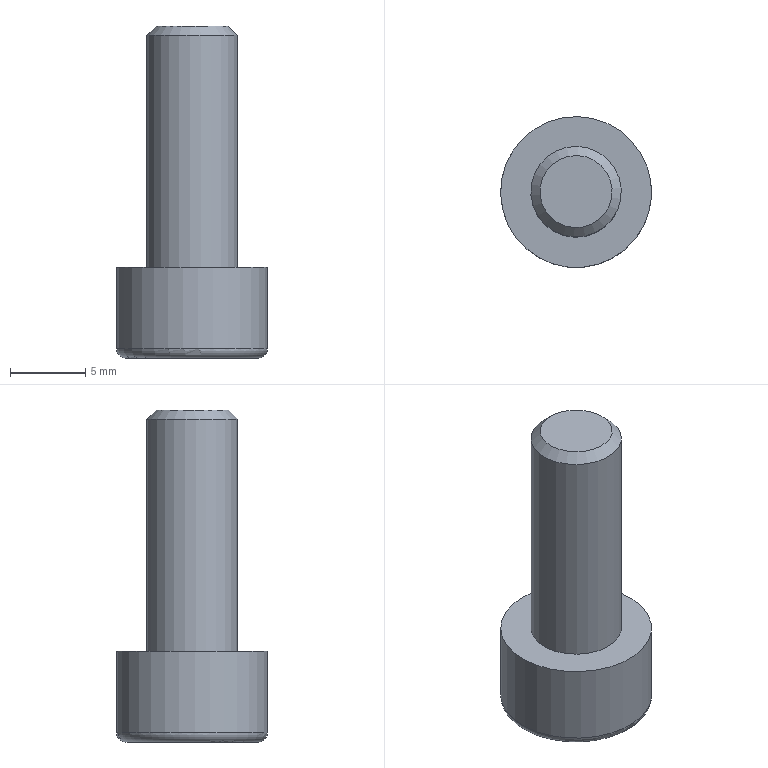Component | NX | SCREW | 1 solid | 14 faces | box 10 x 10 x 22 mm | volume 853 mm3 | plane 10 | cylinder 2 | torus 1 | cone 1 | commonest cylinder face diameters 6 x1 10 x1
STEP:
#1=CARTESIAN_POINT('',(0.,0.,0.));
#2=DIRECTION('',(0.,0.,1.));
#3=DIRECTION('',(1.,0.,0.));
#4=AXIS2_PLACEMENT_3D('',#1,#2,#3);
#5=CARTESIAN_POINT('',(-25.749,-16.598,-131.81));
#6=VERTEX_POINT('',#5);
#7=CARTESIAN_POINT('',(-24.249,-14.,-131.81));
#8=DIRECTION('',(0.,0.,-1.));
#9=DIRECTION('',(-0.5,-0.866,0.));
#10=AXIS2_PLACEMENT_3D('',#7,#8,#9);
#11=CIRCLE('',#10,3.);
#12=CARTESIAN_POINT('',(-24.249,-14.,-147.2));
#13=DIRECTION('',(0.,0.,1.));
#14=DIRECTION('',(0.5,0.866,0.));
#15=AXIS2_PLACEMENT_3D('',#12,#13,#14);
#16=CYLINDRICAL_SURFACE('',#15,3.);
#17=CARTESIAN_POINT('',(9.425,15.39));
#18=DIRECTION('',(-1.,0.));
#19=VECTOR('',#18,1.);
#20=LINE('',#17,#19);
#21=(GEOMETRIC_REPRESENTATION_CONTEXT(2)PARAMETRIC_REPRESENTATION_CONTEXT()REPRESENTATION_CONTEXT('',''));
#22=DEFINITIONAL_REPRESENTATION('',(#20),#21);
#23=PCURVE('',#16,#22);
#24=CARTESIAN_POINT('',(-24.249,-14.,-131.81));
#25=DIRECTION('',(0.,0.,-1.));
#26=DIRECTION('',(-0.5,-0.866,0.));
#27=AXIS2_PLACEMENT_3D('',#24,#25,#26);
#28=CONICAL_SURFACE('',#27,3.,0.7854);
#29=CARTESIAN_POINT('',(0.,0.));
#30=DIRECTION('',(1.,0.));
#31=VECTOR('',#30,1.);
#32=LINE('',#29,#31);
#33=(GEOMETRIC_REPRESENTATION_CONTEXT(2)PARAMETRIC_REPRESENTATION_CONTEXT()REPRESENTATION_CONTEXT('',''));
#34=DEFINITIONAL_REPRESENTATION('',(#32),#33);
#35=PCURVE('',#28,#34);
#36=SURFACE_CURVE('',#11,(#23,#35),.PCURVE_S1.);
#37=EDGE_CURVE('',#6,#6,#36,.T.);
#38=ORIENTED_EDGE('',*,*,#37,.T.);
#39=CARTESIAN_POINT('',(-25.749,-16.598,-147.2));
#40=VERTEX_POINT('',#39);
#41=CARTESIAN_POINT('',(-25.749,-16.598,-147.2));
#42=CARTESIAN_POINT('',(-25.749,-16.598,-131.81));
#43=B_SPLINE_CURVE_WITH_KNOTS('',1,(#41,#42),.UNSPECIFIED.,.F.,.F.,(2,2),(0.,15.39),.PIECEWISE_BEZIER_KNOTS.);
#44=CARTESIAN_POINT('',(3.142,0.));
#45=DIRECTION('',(0.,1.));
#46=VECTOR('',#45,1.);
#47=LINE('',#44,#46);
#48=(GEOMETRIC_REPRESENTATION_CONTEXT(2)PARAMETRIC_REPRESENTATION_CONTEXT()REPRESENTATION_CONTEXT('',''));
#49=DEFINITIONAL_REPRESENTATION('',(#47),#48);
#50=PCURVE('',#16,#49);
#51=CARTESIAN_POINT('',(9.425,0.));
#52=DIRECTION('',(0.,1.));
#53=VECTOR('',#52,1.);
#54=LINE('',#51,#53);
#55=(GEOMETRIC_REPRESENTATION_CONTEXT(2)PARAMETRIC_REPRESENTATION_CONTEXT()REPRESENTATION_CONTEXT('',''));
#56=DEFINITIONAL_REPRESENTATION('',(#54),#55);
#57=PCURVE('',#16,#56);
#58=SEAM_CURVE('',#43,(#50,#57),.PCURVE_S1.);
#59=EDGE_CURVE('',#40,#6,#58,.T.);
#60=ORIENTED_EDGE('',*,*,#59,.F.);
#61=CARTESIAN_POINT('',(-24.249,-14.,-147.2));
#62=DIRECTION('',(0.,0.,-1.));
#63=DIRECTION('',(-0.5,-0.866,0.));
#64=AXIS2_PLACEMENT_3D('',#61,#62,#63);
#65=CIRCLE('',#64,3.);
#66=CARTESIAN_POINT('',(9.425,0.));
#67=DIRECTION('',(-1.,0.));
#68=VECTOR('',#67,1.);
#69=LINE('',#66,#68);
#70=(GEOMETRIC_REPRESENTATION_CONTEXT(2)PARAMETRIC_REPRESENTATION_CONTEXT()REPRESENTATION_CONTEXT('',''));
#71=DEFINITIONAL_REPRESENTATION('',(#69),#70);
#72=PCURVE('',#16,#71);
#73=CARTESIAN_POINT('',(-24.249,-14.,-147.2));
#74=DIRECTION('',(0.,0.,-1.));
#75=DIRECTION('',(-0.5,-0.866,0.));
#76=AXIS2_PLACEMENT_3D('',#73,#74,#75);
#77=PLANE('',#76);
#78=CARTESIAN_POINT('',(0.,0.));
#79=DIRECTION('',(1.,0.));
#80=AXIS2_PLACEMENT_2D('',#78,#79);
#81=CIRCLE('',#80,3.);
#82=(GEOMETRIC_REPRESENTATION_CONTEXT(2)PARAMETRIC_REPRESENTATION_CONTEXT()REPRESENTATION_CONTEXT('',''));
#83=DEFINITIONAL_REPRESENTATION('',(#81),#82);
#84=PCURVE('',#77,#83);
#85=SURFACE_CURVE('',#65,(#72,#84),.PCURVE_S1.);
#86=EDGE_CURVE('',#40,#40,#85,.T.);
#87=ORIENTED_EDGE('',*,*,#86,.F.);
#88=ORIENTED_EDGE('',*,*,#59,.T.);
#89=EDGE_LOOP('',(#38,#60,#87,#88));
#90=FACE_BOUND('',#89,.T.);
#91=ADVANCED_FACE('',(#90),#16,.T.);
#92=CARTESIAN_POINT('',(-25.444,-16.07,-131.2));
#93=VERTEX_POINT('',#92);
#94=CARTESIAN_POINT('',(-24.249,-14.,-131.2));
#95=DIRECTION('',(0.,0.,1.));
#96=DIRECTION('',(-0.5,-0.866,0.));
#97=AXIS2_PLACEMENT_3D('',#94,#95,#96);
#98=CIRCLE('',#97,2.39);
#99=CARTESIAN_POINT('',(-24.249,-14.,-131.2));
#100=DIRECTION('',(0.,0.,-1.));
#101=DIRECTION('',(-0.5,-0.866,0.));
#102=AXIS2_PLACEMENT_3D('',#99,#100,#101);
#103=PLANE('',#102);
#104=CARTESIAN_POINT('',(2.39,0.));
#105=CARTESIAN_POINT('',(2.39,-4.14));
#106=CARTESIAN_POINT('',(-1.195,-2.07));
#107=CARTESIAN_POINT('',(-4.78,-0.));
#108=CARTESIAN_POINT('',(-1.195,2.07));
#109=CARTESIAN_POINT('',(2.39,4.14));
#110=CARTESIAN_POINT('',(2.39,0.));
#111=(BOUNDED_CURVE()B_SPLINE_CURVE(2,(#104,#105,#106,#107,#108,#109,#110),.UNSPECIFIED.,.T.,.F.)B_SPLINE_CURVE_WITH_KNOTS((1,2,2,2,2,1),(-2.094,0.,2.094,4.189,6.283,8.378),.UNSPECIFIED.)CURVE()GEOMETRIC_REPRESENTATION_ITEM()RATIONAL_B_SPLINE_CURVE((1.,0.5,1.,0.5,1.,0.5,1.))REPRESENTATION_ITEM(''));
#112=(GEOMETRIC_REPRESENTATION_CONTEXT(2)PARAMETRIC_REPRESENTATION_CONTEXT()REPRESENTATION_CONTEXT('',''));
#113=DEFINITIONAL_REPRESENTATION('',(#111),#112);
#114=PCURVE('',#103,#113);
#115=CARTESIAN_POINT('',(6.283,-0.61));
#116=DIRECTION('',(-1.,0.));
#117=VECTOR('',#116,1.);
#118=LINE('',#115,#117);
#119=(GEOMETRIC_REPRESENTATION_CONTEXT(2)PARAMETRIC_REPRESENTATION_CONTEXT()REPRESENTATION_CONTEXT('',''));
#120=DEFINITIONAL_REPRESENTATION('',(#118),#119);
#121=PCURVE('',#28,#120);
#122=SURFACE_CURVE('',#98,(#114,#121),.PCURVE_S1.);
#123=EDGE_CURVE('',#93,#93,#122,.T.);
#124=ORIENTED_EDGE('',*,*,#123,.T.);
#125=EDGE_LOOP('',(#124));
#126=FACE_BOUND('',#125,.T.);
#127=ADVANCED_FACE('',(#126),#103,.F.);
#128=CARTESIAN_POINT('',(-26.749,-18.33,-152.6));
#129=VERTEX_POINT('',#128);
#130=CARTESIAN_POINT('',(-24.249,-14.,-152.6));
#131=DIRECTION('',(0.,0.,1.));
#132=DIRECTION('',(-0.5,-0.866,0.));
#133=AXIS2_PLACEMENT_3D('',#130,#131,#132);
#134=CIRCLE('',#133,5.);
#135=CARTESIAN_POINT('',(-24.249,-14.,-153.2));
#136=DIRECTION('',(0.,0.,1.));
#137=DIRECTION('',(0.5,0.866,0.));
#138=AXIS2_PLACEMENT_3D('',#135,#136,#137);
#139=CYLINDRICAL_SURFACE('',#138,5.);
#140=CARTESIAN_POINT('',(3.142,0.6));
#141=DIRECTION('',(1.,0.));
#142=VECTOR('',#141,1.);
#143=LINE('',#140,#142);
#144=(GEOMETRIC_REPRESENTATION_CONTEXT(2)PARAMETRIC_REPRESENTATION_CONTEXT()REPRESENTATION_CONTEXT('',''));
#145=DEFINITIONAL_REPRESENTATION('',(#143),#144);
#146=PCURVE('',#139,#145);
#147=CARTESIAN_POINT('',(-24.249,-14.,-152.6));
#148=DIRECTION('',(0.,0.,-1.));
#149=DIRECTION('',(-0.5,-0.866,0.));
#150=AXIS2_PLACEMENT_3D('',#147,#148,#149);
#151=TOROIDAL_SURFACE('',#150,4.4,0.6);
#152=CARTESIAN_POINT('',(6.283,6.283));
#153=DIRECTION('',(-1.,0.));
#154=VECTOR('',#153,1.);
#155=LINE('',#152,#154);
#156=(GEOMETRIC_REPRESENTATION_CONTEXT(2)PARAMETRIC_REPRESENTATION_CONTEXT()REPRESENTATION_CONTEXT('',''));
#157=DEFINITIONAL_REPRESENTATION('',(#155),#156);
#158=PCURVE('',#151,#157);
#159=SURFACE_CURVE('',#134,(#146,#158),.PCURVE_S1.);
#160=EDGE_CURVE('',#129,#129,#159,.T.);
#161=ORIENTED_EDGE('',*,*,#160,.T.);
#162=CARTESIAN_POINT('',(-26.749,-18.33,-147.2));
#163=VERTEX_POINT('',#162);
#164=CARTESIAN_POINT('',(-26.749,-18.33,-152.6));
#165=CARTESIAN_POINT('',(-26.749,-18.33,-147.2));
#166=B_SPLINE_CURVE_WITH_KNOTS('',1,(#164,#165),.UNSPECIFIED.,.F.,.F.,(2,2),(0.6,6.),.PIECEWISE_BEZIER_KNOTS.);
#167=CARTESIAN_POINT('',(9.425,0.));
#168=DIRECTION('',(0.,1.));
#169=VECTOR('',#168,1.);
#170=LINE('',#167,#169);
#171=(GEOMETRIC_REPRESENTATION_CONTEXT(2)PARAMETRIC_REPRESENTATION_CONTEXT()REPRESENTATION_CONTEXT('',''));
#172=DEFINITIONAL_REPRESENTATION('',(#170),#171);
#173=PCURVE('',#139,#172);
#174=CARTESIAN_POINT('',(3.142,0.));
#175=DIRECTION('',(0.,1.));
#176=VECTOR('',#175,1.);
#177=LINE('',#174,#176);
#178=(GEOMETRIC_REPRESENTATION_CONTEXT(2)PARAMETRIC_REPRESENTATION_CONTEXT()REPRESENTATION_CONTEXT('',''));
#179=DEFINITIONAL_REPRESENTATION('',(#177),#178);
#180=PCURVE('',#139,#179);
#181=SEAM_CURVE('',#166,(#173,#180),.PCURVE_S1.);
#182=EDGE_CURVE('',#129,#163,#181,.T.);
#183=ORIENTED_EDGE('',*,*,#182,.T.);
#184=CARTESIAN_POINT('',(-24.249,-14.,-147.2));
#185=DIRECTION('',(0.,0.,-1.));
#186=DIRECTION('',(-0.5,-0.866,0.));
#187=AXIS2_PLACEMENT_3D('',#184,#185,#186);
#188=CIRCLE('',#187,5.);
#189=CARTESIAN_POINT('',(9.425,6.));
#190=DIRECTION('',(-1.,0.));
#191=VECTOR('',#190,1.);
#192=LINE('',#189,#191);
#193=(GEOMETRIC_REPRESENTATION_CONTEXT(2)PARAMETRIC_REPRESENTATION_CONTEXT()REPRESENTATION_CONTEXT('',''));
#194=DEFINITIONAL_REPRESENTATION('',(#192),#193);
#195=PCURVE('',#139,#194);
#196=CARTESIAN_POINT('',(0.,0.));
#197=DIRECTION('',(1.,0.));
#198=AXIS2_PLACEMENT_2D('',#196,#197);
#199=CIRCLE('',#198,5.);
#200=(GEOMETRIC_REPRESENTATION_CONTEXT(2)PARAMETRIC_REPRESENTATION_CONTEXT()REPRESENTATION_CONTEXT('',''));
#201=DEFINITIONAL_REPRESENTATION('',(#199),#200);
#202=PCURVE('',#77,#201);
#203=SURFACE_CURVE('',#188,(#195,#202),.PCURVE_S1.);
#204=EDGE_CURVE('',#163,#163,#203,.T.);
#205=ORIENTED_EDGE('',*,*,#204,.T.);
#206=ORIENTED_EDGE('',*,*,#182,.F.);
#207=EDGE_LOOP('',(#161,#183,#205,#206));
#208=FACE_BOUND('',#207,.T.);
#209=ADVANCED_FACE('',(#208),#139,.T.);
#210=CARTESIAN_POINT('',(-24.249,-11.113,-153.2));
#211=VERTEX_POINT('',#210);
#212=CARTESIAN_POINT('',(-21.749,-12.557,-153.2));
#213=VERTEX_POINT('',#212);
#214=CARTESIAN_POINT('',(-24.249,-11.113,-153.2));
#215=DIRECTION('',(0.866,-0.5,0.));
#216=VECTOR('',#215,1.);
#217=LINE('',#214,#216);
#218=CARTESIAN_POINT('',(-24.249,-14.,-153.2));
#219=DIRECTION('',(0.,0.,-1.));
#220=DIRECTION('',(-0.5,-0.866,0.));
#221=AXIS2_PLACEMENT_3D('',#218,#219,#220);
#222=PLANE('',#221);
#223=CARTESIAN_POINT('',(-2.5,1.443));
#224=DIRECTION('',(0.,-1.));
#225=VECTOR('',#224,1.);
#226=LINE('',#223,#225);
#227=(GEOMETRIC_REPRESENTATION_CONTEXT(2)PARAMETRIC_REPRESENTATION_CONTEXT()REPRESENTATION_CONTEXT('',''));
#228=DEFINITIONAL_REPRESENTATION('',(#226),#227);
#229=PCURVE('',#222,#228);
#230=CARTESIAN_POINT('',(-24.249,-11.113,-150.2));
#231=DIRECTION('',(0.5,0.866,0.));
#232=DIRECTION('',(0.,0.,-1.));
#233=AXIS2_PLACEMENT_3D('',#230,#231,#232);
#234=PLANE('',#233);
#235=CARTESIAN_POINT('',(3.,0.));
#236=DIRECTION('',(0.,-1.));
#237=VECTOR('',#236,1.);
#238=LINE('',#235,#237);
#239=(GEOMETRIC_REPRESENTATION_CONTEXT(2)PARAMETRIC_REPRESENTATION_CONTEXT()REPRESENTATION_CONTEXT('',''));
#240=DEFINITIONAL_REPRESENTATION('',(#238),#239);
#241=PCURVE('',#234,#240);
#242=SURFACE_CURVE('',#217,(#229,#241),.PCURVE_S1.);
#243=EDGE_CURVE('',#211,#213,#242,.T.);
#244=ORIENTED_EDGE('',*,*,#243,.F.);
#245=CARTESIAN_POINT('',(-26.749,-12.557,-153.2));
#246=VERTEX_POINT('',#245);
#247=CARTESIAN_POINT('',(-26.749,-12.557,-153.2));
#248=DIRECTION('',(0.866,0.5,0.));
#249=VECTOR('',#248,1.);
#250=LINE('',#247,#249);
#251=CARTESIAN_POINT('',(-0.,2.887));
#252=DIRECTION('',(-0.866,-0.5));
#253=VECTOR('',#252,1.);
#254=LINE('',#251,#253);
#255=(GEOMETRIC_REPRESENTATION_CONTEXT(2)PARAMETRIC_REPRESENTATION_CONTEXT()REPRESENTATION_CONTEXT('',''));
#256=DEFINITIONAL_REPRESENTATION('',(#254),#255);
#257=PCURVE('',#222,#256);
#258=CARTESIAN_POINT('',(-26.749,-12.557,-150.2));
#259=DIRECTION('',(-0.5,0.866,0.));
#260=DIRECTION('',(0.866,0.5,0.));
#261=AXIS2_PLACEMENT_3D('',#258,#259,#260);
#262=PLANE('',#261);
#263=CARTESIAN_POINT('',(0.,3.));
#264=DIRECTION('',(1.,0.));
#265=VECTOR('',#264,1.);
#266=LINE('',#263,#265);
#267=(GEOMETRIC_REPRESENTATION_CONTEXT(2)PARAMETRIC_REPRESENTATION_CONTEXT()REPRESENTATION_CONTEXT('',''));
#268=DEFINITIONAL_REPRESENTATION('',(#266),#267);
#269=PCURVE('',#262,#268);
#270=SURFACE_CURVE('',#250,(#257,#269),.PCURVE_S1.);
#271=EDGE_CURVE('',#246,#211,#270,.T.);
#272=ORIENTED_EDGE('',*,*,#271,.F.);
#273=CARTESIAN_POINT('',(-26.749,-15.443,-153.2));
#274=VERTEX_POINT('',#273);
#275=CARTESIAN_POINT('',(-26.749,-15.443,-153.2));
#276=DIRECTION('',(-0.,1.,0.));
#277=VECTOR('',#276,1.);
#278=LINE('',#275,#277);
#279=CARTESIAN_POINT('',(2.5,1.443));
#280=DIRECTION('',(-0.866,0.5));
#281=VECTOR('',#280,1.);
#282=LINE('',#279,#281);
#283=(GEOMETRIC_REPRESENTATION_CONTEXT(2)PARAMETRIC_REPRESENTATION_CONTEXT()REPRESENTATION_CONTEXT('',''));
#284=DEFINITIONAL_REPRESENTATION('',(#282),#283);
#285=PCURVE('',#222,#284);
#286=CARTESIAN_POINT('',(-26.749,-15.443,-150.2));
#287=DIRECTION('',(-1.,-0.,0.));
#288=DIRECTION('',(-0.,1.,0.));
#289=AXIS2_PLACEMENT_3D('',#286,#287,#288);
#290=PLANE('',#289);
#291=CARTESIAN_POINT('',(0.,3.));
#292=DIRECTION('',(1.,0.));
#293=VECTOR('',#292,1.);
#294=LINE('',#291,#293);
#295=(GEOMETRIC_REPRESENTATION_CONTEXT(2)PARAMETRIC_REPRESENTATION_CONTEXT()REPRESENTATION_CONTEXT('',''));
#296=DEFINITIONAL_REPRESENTATION('',(#294),#295);
#297=PCURVE('',#290,#296);
#298=SURFACE_CURVE('',#278,(#285,#297),.PCURVE_S1.);
#299=EDGE_CURVE('',#274,#246,#298,.T.);
#300=ORIENTED_EDGE('',*,*,#299,.F.);
#301=CARTESIAN_POINT('',(-24.249,-16.887,-153.2));
#302=VERTEX_POINT('',#301);
#303=CARTESIAN_POINT('',(-24.249,-16.887,-153.2));
#304=DIRECTION('',(-0.866,0.5,0.));
#305=VECTOR('',#304,1.);
#306=LINE('',#303,#305);
#307=CARTESIAN_POINT('',(2.5,-1.443));
#308=DIRECTION('',(0.,1.));
#309=VECTOR('',#308,1.);
#310=LINE('',#307,#309);
#311=(GEOMETRIC_REPRESENTATION_CONTEXT(2)PARAMETRIC_REPRESENTATION_CONTEXT()REPRESENTATION_CONTEXT('',''));
#312=DEFINITIONAL_REPRESENTATION('',(#310),#311);
#313=PCURVE('',#222,#312);
#314=CARTESIAN_POINT('',(-24.249,-16.887,-150.2));
#315=DIRECTION('',(-0.5,-0.866,0.));
#316=DIRECTION('',(0.,0.,1.));
#317=AXIS2_PLACEMENT_3D('',#314,#315,#316);
#318=PLANE('',#317);
#319=CARTESIAN_POINT('',(-3.,0.));
#320=DIRECTION('',(0.,1.));
#321=VECTOR('',#320,1.);
#322=LINE('',#319,#321);
#323=(GEOMETRIC_REPRESENTATION_CONTEXT(2)PARAMETRIC_REPRESENTATION_CONTEXT()REPRESENTATION_CONTEXT('',''));
#324=DEFINITIONAL_REPRESENTATION('',(#322),#323);
#325=PCURVE('',#318,#324);
#326=SURFACE_CURVE('',#306,(#313,#325),.PCURVE_S1.);
#327=EDGE_CURVE('',#302,#274,#326,.T.);
#328=ORIENTED_EDGE('',*,*,#327,.F.);
#329=CARTESIAN_POINT('',(-21.749,-15.443,-153.2));
#330=VERTEX_POINT('',#329);
#331=CARTESIAN_POINT('',(-21.749,-15.443,-153.2));
#332=DIRECTION('',(-0.866,-0.5,0.));
#333=VECTOR('',#332,1.);
#334=LINE('',#331,#333);
#335=CARTESIAN_POINT('',(-0.,-2.887));
#336=DIRECTION('',(0.866,0.5));
#337=VECTOR('',#336,1.);
#338=LINE('',#335,#337);
#339=(GEOMETRIC_REPRESENTATION_CONTEXT(2)PARAMETRIC_REPRESENTATION_CONTEXT()REPRESENTATION_CONTEXT('',''));
#340=DEFINITIONAL_REPRESENTATION('',(#338),#339);
#341=PCURVE('',#222,#340);
#342=CARTESIAN_POINT('',(-21.749,-15.443,-150.2));
#343=DIRECTION('',(0.5,-0.866,0.));
#344=DIRECTION('',(-0.866,-0.5,0.));
#345=AXIS2_PLACEMENT_3D('',#342,#343,#344);
#346=PLANE('',#345);
#347=CARTESIAN_POINT('',(0.,3.));
#348=DIRECTION('',(1.,0.));
#349=VECTOR('',#348,1.);
#350=LINE('',#347,#349);
#351=(GEOMETRIC_REPRESENTATION_CONTEXT(2)PARAMETRIC_REPRESENTATION_CONTEXT()REPRESENTATION_CONTEXT('',''));
#352=DEFINITIONAL_REPRESENTATION('',(#350),#351);
#353=PCURVE('',#346,#352);
#354=SURFACE_CURVE('',#334,(#341,#353),.PCURVE_S1.);
#355=EDGE_CURVE('',#330,#302,#354,.T.);
#356=ORIENTED_EDGE('',*,*,#355,.F.);
#357=CARTESIAN_POINT('',(-21.749,-12.557,-153.2));
#358=DIRECTION('',(0.,-1.,0.));
#359=VECTOR('',#358,1.);
#360=LINE('',#357,#359);
#361=CARTESIAN_POINT('',(-2.5,-1.443));
#362=DIRECTION('',(0.866,-0.5));
#363=VECTOR('',#362,1.);
#364=LINE('',#361,#363);
#365=(GEOMETRIC_REPRESENTATION_CONTEXT(2)PARAMETRIC_REPRESENTATION_CONTEXT()REPRESENTATION_CONTEXT('',''));
#366=DEFINITIONAL_REPRESENTATION('',(#364),#365);
#367=PCURVE('',#222,#366);
#368=CARTESIAN_POINT('',(-21.749,-12.557,-150.2));
#369=DIRECTION('',(1.,0.,0.));
#370=DIRECTION('',(0.,-1.,0.));
#371=AXIS2_PLACEMENT_3D('',#368,#369,#370);
#372=PLANE('',#371);
#373=CARTESIAN_POINT('',(0.,3.));
#374=DIRECTION('',(1.,0.));
#375=VECTOR('',#374,1.);
#376=LINE('',#373,#375);
#377=(GEOMETRIC_REPRESENTATION_CONTEXT(2)PARAMETRIC_REPRESENTATION_CONTEXT()REPRESENTATION_CONTEXT('',''));
#378=DEFINITIONAL_REPRESENTATION('',(#376),#377);
#379=PCURVE('',#372,#378);
#380=SURFACE_CURVE('',#360,(#367,#379),.PCURVE_S1.);
#381=EDGE_CURVE('',#213,#330,#380,.T.);
#382=ORIENTED_EDGE('',*,*,#381,.F.);
#383=EDGE_LOOP('',(#244,#272,#300,#328,#356,#382));
#384=FACE_BOUND('',#383,.T.);
#385=CARTESIAN_POINT('',(-26.449,-17.811,-153.2));
#386=VERTEX_POINT('',#385);
#387=CARTESIAN_POINT('',(-24.249,-14.,-153.2));
#388=DIRECTION('',(0.,0.,-1.));
#389=DIRECTION('',(-0.5,-0.866,0.));
#390=AXIS2_PLACEMENT_3D('',#387,#388,#389);
#391=CIRCLE('',#390,4.4);
#392=CARTESIAN_POINT('',(0.,0.));
#393=DIRECTION('',(1.,0.));
#394=AXIS2_PLACEMENT_2D('',#392,#393);
#395=CIRCLE('',#394,4.4);
#396=(GEOMETRIC_REPRESENTATION_CONTEXT(2)PARAMETRIC_REPRESENTATION_CONTEXT()REPRESENTATION_CONTEXT('',''));
#397=DEFINITIONAL_REPRESENTATION('',(#395),#396);
#398=PCURVE('',#222,#397);
#399=CARTESIAN_POINT('',(0.,7.854));
#400=DIRECTION('',(1.,0.));
#401=VECTOR('',#400,1.);
#402=LINE('',#399,#401);
#403=(GEOMETRIC_REPRESENTATION_CONTEXT(2)PARAMETRIC_REPRESENTATION_CONTEXT()REPRESENTATION_CONTEXT('',''));
#404=DEFINITIONAL_REPRESENTATION('',(#402),#403);
#405=PCURVE('',#151,#404);
#406=SURFACE_CURVE('',#391,(#398,#405),.PCURVE_S1.);
#407=EDGE_CURVE('',#386,#386,#406,.T.);
#408=ORIENTED_EDGE('',*,*,#407,.T.);
#409=EDGE_LOOP('',(#408));
#410=FACE_BOUND('',#409,.T.);
#411=ADVANCED_FACE('',(#384,#410),#222,.T.);
#412=ORIENTED_EDGE('',*,*,#86,.T.);
#413=EDGE_LOOP('',(#412));
#414=FACE_BOUND('',#413,.T.);
#415=ORIENTED_EDGE('',*,*,#204,.F.);
#416=EDGE_LOOP('',(#415));
#417=FACE_BOUND('',#416,.T.);
#418=ADVANCED_FACE('',(#414,#417),#77,.F.);
#419=ORIENTED_EDGE('',*,*,#160,.F.);
#420=CARTESIAN_POINT('',(-26.749,-18.33,-152.6));
#421=CARTESIAN_POINT('',(-26.749,-18.33,-152.76));
#422=CARTESIAN_POINT('',(-26.723,-18.286,-152.917));
#423=CARTESIAN_POINT('',(-26.674,-18.201,-153.051));
#424=CARTESIAN_POINT('',(-26.607,-18.085,-153.149));
#425=CARTESIAN_POINT('',(-26.529,-17.949,-153.2));
#426=CARTESIAN_POINT('',(-26.449,-17.811,-153.2));
#427=(BOUNDED_CURVE()B_SPLINE_CURVE(6,(#420,#421,#422,#423,#424,#425,#426),.UNSPECIFIED.,.F.,.F.)B_SPLINE_CURVE_WITH_KNOTS((7,7),(0.,1.571),.PIECEWISE_BEZIER_KNOTS.)CURVE()GEOMETRIC_REPRESENTATION_ITEM()RATIONAL_B_SPLINE_CURVE((1.031,1.01,0.9979,0.994,0.9979,1.01,1.031))REPRESENTATION_ITEM(''));
#428=CARTESIAN_POINT('',(6.283,6.283));
#429=DIRECTION('',(0.,1.));
#430=VECTOR('',#429,1.);
#431=LINE('',#428,#430);
#432=(GEOMETRIC_REPRESENTATION_CONTEXT(2)PARAMETRIC_REPRESENTATION_CONTEXT()REPRESENTATION_CONTEXT('',''));
#433=DEFINITIONAL_REPRESENTATION('',(#431),#432);
#434=PCURVE('',#151,#433);
#435=CARTESIAN_POINT('',(0.,6.283));
#436=DIRECTION('',(0.,1.));
#437=VECTOR('',#436,1.);
#438=LINE('',#435,#437);
#439=(GEOMETRIC_REPRESENTATION_CONTEXT(2)PARAMETRIC_REPRESENTATION_CONTEXT()REPRESENTATION_CONTEXT('',''));
#440=DEFINITIONAL_REPRESENTATION('',(#438),#439);
#441=PCURVE('',#151,#440);
#442=SEAM_CURVE('',#427,(#434,#441),.PCURVE_S1.);
#443=EDGE_CURVE('',#129,#386,#442,.T.);
#444=ORIENTED_EDGE('',*,*,#443,.T.);
#445=ORIENTED_EDGE('',*,*,#407,.F.);
#446=ORIENTED_EDGE('',*,*,#443,.F.);
#447=EDGE_LOOP('',(#419,#444,#445,#446));
#448=FACE_BOUND('',#447,.T.);
#449=ADVANCED_FACE('',(#448),#151,.T.);
#450=ORIENTED_EDGE('',*,*,#123,.F.);
#451=CARTESIAN_POINT('',(-25.444,-16.07,-131.2));
#452=CARTESIAN_POINT('',(-25.749,-16.598,-131.81));
#453=B_SPLINE_CURVE_WITH_KNOTS('',1,(#451,#452),.UNSPECIFIED.,.F.,.F.,(2,2),(-0.8627,0.),.PIECEWISE_BEZIER_KNOTS.);
#454=CARTESIAN_POINT('',(6.283,0.));
#455=DIRECTION('',(0.,1.));
#456=VECTOR('',#455,1.);
#457=LINE('',#454,#456);
#458=(GEOMETRIC_REPRESENTATION_CONTEXT(2)PARAMETRIC_REPRESENTATION_CONTEXT()REPRESENTATION_CONTEXT('',''));
#459=DEFINITIONAL_REPRESENTATION('',(#457),#458);
#460=PCURVE('',#28,#459);
#461=CARTESIAN_POINT('',(0.,0.));
#462=DIRECTION('',(0.,1.));
#463=VECTOR('',#462,1.);
#464=LINE('',#461,#463);
#465=(GEOMETRIC_REPRESENTATION_CONTEXT(2)PARAMETRIC_REPRESENTATION_CONTEXT()REPRESENTATION_CONTEXT('',''));
#466=DEFINITIONAL_REPRESENTATION('',(#464),#465);
#467=PCURVE('',#28,#466);
#468=SEAM_CURVE('',#453,(#460,#467),.PCURVE_S1.);
#469=EDGE_CURVE('',#93,#6,#468,.T.);
#470=ORIENTED_EDGE('',*,*,#469,.T.);
#471=ORIENTED_EDGE('',*,*,#37,.F.);
#472=ORIENTED_EDGE('',*,*,#469,.F.);
#473=EDGE_LOOP('',(#450,#470,#471,#472));
#474=FACE_BOUND('',#473,.T.);
#475=ADVANCED_FACE('',(#474),#28,.T.);
#476=ORIENTED_EDGE('',*,*,#243,.T.);
#477=CARTESIAN_POINT('',(-21.749,-12.557,-150.2));
#478=VERTEX_POINT('',#477);
#479=CARTESIAN_POINT('',(-21.749,-12.557,-150.2));
#480=DIRECTION('',(0.,0.,1.));
#481=VECTOR('',#480,1.);
#482=LINE('',#479,#481);
#483=CARTESIAN_POINT('',(0.,-2.887));
#484=DIRECTION('',(-1.,0.));
#485=VECTOR('',#484,1.);
#486=LINE('',#483,#485);
#487=(GEOMETRIC_REPRESENTATION_CONTEXT(2)PARAMETRIC_REPRESENTATION_CONTEXT()REPRESENTATION_CONTEXT('',''));
#488=DEFINITIONAL_REPRESENTATION('',(#486),#487);
#489=PCURVE('',#234,#488);
#490=CARTESIAN_POINT('',(0.,0.));
#491=DIRECTION('',(0.,-1.));
#492=VECTOR('',#491,1.);
#493=LINE('',#490,#492);
#494=(GEOMETRIC_REPRESENTATION_CONTEXT(2)PARAMETRIC_REPRESENTATION_CONTEXT()REPRESENTATION_CONTEXT('',''));
#495=DEFINITIONAL_REPRESENTATION('',(#493),#494);
#496=PCURVE('',#372,#495);
#497=SURFACE_CURVE('',#482,(#489,#496),.PCURVE_S1.);
#498=EDGE_CURVE('',#213,#478,#497,.T.);
#499=ORIENTED_EDGE('',*,*,#498,.T.);
#500=CARTESIAN_POINT('',(-24.249,-11.113,-150.2));
#501=VERTEX_POINT('',#500);
#502=CARTESIAN_POINT('',(-24.249,-11.113,-150.2));
#503=DIRECTION('',(-0.866,0.5,0.));
#504=VECTOR('',#503,1.);
#505=LINE('',#502,#504);
#506=CARTESIAN_POINT('',(0.,0.));
#507=DIRECTION('',(0.,1.));
#508=VECTOR('',#507,1.);
#509=LINE('',#506,#508);
#510=(GEOMETRIC_REPRESENTATION_CONTEXT(2)PARAMETRIC_REPRESENTATION_CONTEXT()REPRESENTATION_CONTEXT('',''));
#511=DEFINITIONAL_REPRESENTATION('',(#509),#510);
#512=PCURVE('',#234,#511);
#513=CARTESIAN_POINT('',(-24.249,-14.,-150.2));
#514=DIRECTION('',(0.,0.,-1.));
#515=DIRECTION('',(-0.5,-0.866,0.));
#516=AXIS2_PLACEMENT_3D('',#513,#514,#515);
#517=PLANE('',#516);
#518=CARTESIAN_POINT('',(-2.5,1.443));
#519=DIRECTION('',(0.,1.));
#520=VECTOR('',#519,1.);
#521=LINE('',#518,#520);
#522=(GEOMETRIC_REPRESENTATION_CONTEXT(2)PARAMETRIC_REPRESENTATION_CONTEXT()REPRESENTATION_CONTEXT('',''));
#523=DEFINITIONAL_REPRESENTATION('',(#521),#522);
#524=PCURVE('',#517,#523);
#525=SURFACE_CURVE('',#505,(#512,#524),.PCURVE_S1.);
#526=EDGE_CURVE('',#478,#501,#525,.T.);
#527=ORIENTED_EDGE('',*,*,#526,.T.);
#528=CARTESIAN_POINT('',(-24.249,-11.113,-150.2));
#529=DIRECTION('',(0.,0.,1.));
#530=VECTOR('',#529,1.);
#531=LINE('',#528,#530);
#532=CARTESIAN_POINT('',(0.,0.));
#533=DIRECTION('',(-1.,0.));
#534=VECTOR('',#533,1.);
#535=LINE('',#532,#534);
#536=(GEOMETRIC_REPRESENTATION_CONTEXT(2)PARAMETRIC_REPRESENTATION_CONTEXT()REPRESENTATION_CONTEXT('',''));
#537=DEFINITIONAL_REPRESENTATION('',(#535),#536);
#538=PCURVE('',#234,#537);
#539=CARTESIAN_POINT('',(2.887,0.));
#540=DIRECTION('',(0.,-1.));
#541=VECTOR('',#540,1.);
#542=LINE('',#539,#541);
#543=(GEOMETRIC_REPRESENTATION_CONTEXT(2)PARAMETRIC_REPRESENTATION_CONTEXT()REPRESENTATION_CONTEXT('',''));
#544=DEFINITIONAL_REPRESENTATION('',(#542),#543);
#545=PCURVE('',#262,#544);
#546=SURFACE_CURVE('',#531,(#538,#545),.PCURVE_S1.);
#547=EDGE_CURVE('',#211,#501,#546,.T.);
#548=ORIENTED_EDGE('',*,*,#547,.F.);
#549=EDGE_LOOP('',(#476,#499,#527,#548));
#550=FACE_BOUND('',#549,.T.);
#551=ADVANCED_FACE('',(#550),#234,.F.);
#552=ORIENTED_EDGE('',*,*,#381,.T.);
#553=CARTESIAN_POINT('',(-21.749,-15.443,-150.2));
#554=VERTEX_POINT('',#553);
#555=CARTESIAN_POINT('',(-21.749,-15.443,-150.2));
#556=DIRECTION('',(0.,0.,1.));
#557=VECTOR('',#556,1.);
#558=LINE('',#555,#557);
#559=CARTESIAN_POINT('',(2.887,0.));
#560=DIRECTION('',(0.,-1.));
#561=VECTOR('',#560,1.);
#562=LINE('',#559,#561);
#563=(GEOMETRIC_REPRESENTATION_CONTEXT(2)PARAMETRIC_REPRESENTATION_CONTEXT()REPRESENTATION_CONTEXT('',''));
#564=DEFINITIONAL_REPRESENTATION('',(#562),#563);
#565=PCURVE('',#372,#564);
#566=CARTESIAN_POINT('',(0.,0.));
#567=DIRECTION('',(0.,-1.));
#568=VECTOR('',#567,1.);
#569=LINE('',#566,#568);
#570=(GEOMETRIC_REPRESENTATION_CONTEXT(2)PARAMETRIC_REPRESENTATION_CONTEXT()REPRESENTATION_CONTEXT('',''));
#571=DEFINITIONAL_REPRESENTATION('',(#569),#570);
#572=PCURVE('',#346,#571);
#573=SURFACE_CURVE('',#558,(#565,#572),.PCURVE_S1.);
#574=EDGE_CURVE('',#330,#554,#573,.T.);
#575=ORIENTED_EDGE('',*,*,#574,.T.);
#576=CARTESIAN_POINT('',(-21.749,-12.557,-150.2));
#577=DIRECTION('',(-0.,1.,0.));
#578=VECTOR('',#577,1.);
#579=LINE('',#576,#578);
#580=CARTESIAN_POINT('',(0.,0.));
#581=DIRECTION('',(-1.,0.));
#582=VECTOR('',#581,1.);
#583=LINE('',#580,#582);
#584=(GEOMETRIC_REPRESENTATION_CONTEXT(2)PARAMETRIC_REPRESENTATION_CONTEXT()REPRESENTATION_CONTEXT('',''));
#585=DEFINITIONAL_REPRESENTATION('',(#583),#584);
#586=PCURVE('',#372,#585);
#587=CARTESIAN_POINT('',(-2.5,-1.443));
#588=DIRECTION('',(-0.866,0.5));
#589=VECTOR('',#588,1.);
#590=LINE('',#587,#589);
#591=(GEOMETRIC_REPRESENTATION_CONTEXT(2)PARAMETRIC_REPRESENTATION_CONTEXT()REPRESENTATION_CONTEXT('',''));
#592=DEFINITIONAL_REPRESENTATION('',(#590),#591);
#593=PCURVE('',#517,#592);
#594=SURFACE_CURVE('',#579,(#586,#593),.PCURVE_S1.);
#595=EDGE_CURVE('',#554,#478,#594,.T.);
#596=ORIENTED_EDGE('',*,*,#595,.T.);
#597=ORIENTED_EDGE('',*,*,#498,.F.);
#598=EDGE_LOOP('',(#552,#575,#596,#597));
#599=FACE_BOUND('',#598,.T.);
#600=ADVANCED_FACE('',(#599),#372,.F.);
#601=ORIENTED_EDGE('',*,*,#355,.T.);
#602=CARTESIAN_POINT('',(-24.249,-16.887,-150.2));
#603=VERTEX_POINT('',#602);
#604=CARTESIAN_POINT('',(-24.249,-16.887,-150.2));
#605=DIRECTION('',(0.,0.,1.));
#606=VECTOR('',#605,1.);
#607=LINE('',#604,#606);
#608=CARTESIAN_POINT('',(2.887,0.));
#609=DIRECTION('',(0.,-1.));
#610=VECTOR('',#609,1.);
#611=LINE('',#608,#610);
#612=(GEOMETRIC_REPRESENTATION_CONTEXT(2)PARAMETRIC_REPRESENTATION_CONTEXT()REPRESENTATION_CONTEXT('',''));
#613=DEFINITIONAL_REPRESENTATION('',(#611),#612);
#614=PCURVE('',#346,#613);
#615=CARTESIAN_POINT('',(0.,0.));
#616=DIRECTION('',(1.,0.));
#617=VECTOR('',#616,1.);
#618=LINE('',#615,#617);
#619=(GEOMETRIC_REPRESENTATION_CONTEXT(2)PARAMETRIC_REPRESENTATION_CONTEXT()REPRESENTATION_CONTEXT('',''));
#620=DEFINITIONAL_REPRESENTATION('',(#618),#619);
#621=PCURVE('',#318,#620);
#622=SURFACE_CURVE('',#607,(#614,#621),.PCURVE_S1.);
#623=EDGE_CURVE('',#302,#603,#622,.T.);
#624=ORIENTED_EDGE('',*,*,#623,.T.);
#625=CARTESIAN_POINT('',(-21.749,-15.443,-150.2));
#626=DIRECTION('',(0.866,0.5,0.));
#627=VECTOR('',#626,1.);
#628=LINE('',#625,#627);
#629=CARTESIAN_POINT('',(0.,0.));
#630=DIRECTION('',(-1.,0.));
#631=VECTOR('',#630,1.);
#632=LINE('',#629,#631);
#633=(GEOMETRIC_REPRESENTATION_CONTEXT(2)PARAMETRIC_REPRESENTATION_CONTEXT()REPRESENTATION_CONTEXT('',''));
#634=DEFINITIONAL_REPRESENTATION('',(#632),#633);
#635=PCURVE('',#346,#634);
#636=CARTESIAN_POINT('',(-0.,-2.887));
#637=DIRECTION('',(-0.866,-0.5));
#638=VECTOR('',#637,1.);
#639=LINE('',#636,#638);
#640=(GEOMETRIC_REPRESENTATION_CONTEXT(2)PARAMETRIC_REPRESENTATION_CONTEXT()REPRESENTATION_CONTEXT('',''));
#641=DEFINITIONAL_REPRESENTATION('',(#639),#640);
#642=PCURVE('',#517,#641);
#643=SURFACE_CURVE('',#628,(#635,#642),.PCURVE_S1.);
#644=EDGE_CURVE('',#603,#554,#643,.T.);
#645=ORIENTED_EDGE('',*,*,#644,.T.);
#646=ORIENTED_EDGE('',*,*,#574,.F.);
#647=EDGE_LOOP('',(#601,#624,#645,#646));
#648=FACE_BOUND('',#647,.T.);
#649=ADVANCED_FACE('',(#648),#346,.F.);
#650=ORIENTED_EDGE('',*,*,#327,.T.);
#651=CARTESIAN_POINT('',(-26.749,-15.443,-150.2));
#652=VERTEX_POINT('',#651);
#653=CARTESIAN_POINT('',(-26.749,-15.443,-150.2));
#654=DIRECTION('',(0.,0.,1.));
#655=VECTOR('',#654,1.);
#656=LINE('',#653,#655);
#657=CARTESIAN_POINT('',(0.,2.887));
#658=DIRECTION('',(1.,0.));
#659=VECTOR('',#658,1.);
#660=LINE('',#657,#659);
#661=(GEOMETRIC_REPRESENTATION_CONTEXT(2)PARAMETRIC_REPRESENTATION_CONTEXT()REPRESENTATION_CONTEXT('',''));
#662=DEFINITIONAL_REPRESENTATION('',(#660),#661);
#663=PCURVE('',#318,#662);
#664=CARTESIAN_POINT('',(0.,0.));
#665=DIRECTION('',(0.,-1.));
#666=VECTOR('',#665,1.);
#667=LINE('',#664,#666);
#668=(GEOMETRIC_REPRESENTATION_CONTEXT(2)PARAMETRIC_REPRESENTATION_CONTEXT()REPRESENTATION_CONTEXT('',''));
#669=DEFINITIONAL_REPRESENTATION('',(#667),#668);
#670=PCURVE('',#290,#669);
#671=SURFACE_CURVE('',#656,(#663,#670),.PCURVE_S1.);
#672=EDGE_CURVE('',#274,#652,#671,.T.);
#673=ORIENTED_EDGE('',*,*,#672,.T.);
#674=CARTESIAN_POINT('',(-24.249,-16.887,-150.2));
#675=DIRECTION('',(0.866,-0.5,0.));
#676=VECTOR('',#675,1.);
#677=LINE('',#674,#676);
#678=CARTESIAN_POINT('',(0.,0.));
#679=DIRECTION('',(0.,-1.));
#680=VECTOR('',#679,1.);
#681=LINE('',#678,#680);
#682=(GEOMETRIC_REPRESENTATION_CONTEXT(2)PARAMETRIC_REPRESENTATION_CONTEXT()REPRESENTATION_CONTEXT('',''));
#683=DEFINITIONAL_REPRESENTATION('',(#681),#682);
#684=PCURVE('',#318,#683);
#685=CARTESIAN_POINT('',(2.5,-1.443));
#686=DIRECTION('',(0.,-1.));
#687=VECTOR('',#686,1.);
#688=LINE('',#685,#687);
#689=(GEOMETRIC_REPRESENTATION_CONTEXT(2)PARAMETRIC_REPRESENTATION_CONTEXT()REPRESENTATION_CONTEXT('',''));
#690=DEFINITIONAL_REPRESENTATION('',(#688),#689);
#691=PCURVE('',#517,#690);
#692=SURFACE_CURVE('',#677,(#684,#691),.PCURVE_S1.);
#693=EDGE_CURVE('',#652,#603,#692,.T.);
#694=ORIENTED_EDGE('',*,*,#693,.T.);
#695=ORIENTED_EDGE('',*,*,#623,.F.);
#696=EDGE_LOOP('',(#650,#673,#694,#695));
#697=FACE_BOUND('',#696,.T.);
#698=ADVANCED_FACE('',(#697),#318,.F.);
#699=ORIENTED_EDGE('',*,*,#299,.T.);
#700=CARTESIAN_POINT('',(-26.749,-12.557,-150.2));
#701=VERTEX_POINT('',#700);
#702=CARTESIAN_POINT('',(-26.749,-12.557,-150.2));
#703=DIRECTION('',(0.,0.,1.));
#704=VECTOR('',#703,1.);
#705=LINE('',#702,#704);
#706=CARTESIAN_POINT('',(2.887,0.));
#707=DIRECTION('',(0.,-1.));
#708=VECTOR('',#707,1.);
#709=LINE('',#706,#708);
#710=(GEOMETRIC_REPRESENTATION_CONTEXT(2)PARAMETRIC_REPRESENTATION_CONTEXT()REPRESENTATION_CONTEXT('',''));
#711=DEFINITIONAL_REPRESENTATION('',(#709),#710);
#712=PCURVE('',#290,#711);
#713=CARTESIAN_POINT('',(0.,0.));
#714=DIRECTION('',(0.,-1.));
#715=VECTOR('',#714,1.);
#716=LINE('',#713,#715);
#717=(GEOMETRIC_REPRESENTATION_CONTEXT(2)PARAMETRIC_REPRESENTATION_CONTEXT()REPRESENTATION_CONTEXT('',''));
#718=DEFINITIONAL_REPRESENTATION('',(#716),#717);
#719=PCURVE('',#262,#718);
#720=SURFACE_CURVE('',#705,(#712,#719),.PCURVE_S1.);
#721=EDGE_CURVE('',#246,#701,#720,.T.);
#722=ORIENTED_EDGE('',*,*,#721,.T.);
#723=CARTESIAN_POINT('',(-26.749,-15.443,-150.2));
#724=DIRECTION('',(0.,-1.,0.));
#725=VECTOR('',#724,1.);
#726=LINE('',#723,#725);
#727=CARTESIAN_POINT('',(0.,0.));
#728=DIRECTION('',(-1.,0.));
#729=VECTOR('',#728,1.);
#730=LINE('',#727,#729);
#731=(GEOMETRIC_REPRESENTATION_CONTEXT(2)PARAMETRIC_REPRESENTATION_CONTEXT()REPRESENTATION_CONTEXT('',''));
#732=DEFINITIONAL_REPRESENTATION('',(#730),#731);
#733=PCURVE('',#290,#732);
#734=CARTESIAN_POINT('',(2.5,1.443));
#735=DIRECTION('',(0.866,-0.5));
#736=VECTOR('',#735,1.);
#737=LINE('',#734,#736);
#738=(GEOMETRIC_REPRESENTATION_CONTEXT(2)PARAMETRIC_REPRESENTATION_CONTEXT()REPRESENTATION_CONTEXT('',''));
#739=DEFINITIONAL_REPRESENTATION('',(#737),#738);
#740=PCURVE('',#517,#739);
#741=SURFACE_CURVE('',#726,(#733,#740),.PCURVE_S1.);
#742=EDGE_CURVE('',#701,#652,#741,.T.);
#743=ORIENTED_EDGE('',*,*,#742,.T.);
#744=ORIENTED_EDGE('',*,*,#672,.F.);
#745=EDGE_LOOP('',(#699,#722,#743,#744));
#746=FACE_BOUND('',#745,.T.);
#747=ADVANCED_FACE('',(#746),#290,.F.);
#748=ORIENTED_EDGE('',*,*,#271,.T.);
#749=ORIENTED_EDGE('',*,*,#547,.T.);
#750=CARTESIAN_POINT('',(-26.749,-12.557,-150.2));
#751=DIRECTION('',(-0.866,-0.5,0.));
#752=VECTOR('',#751,1.);
#753=LINE('',#750,#752);
#754=CARTESIAN_POINT('',(0.,0.));
#755=DIRECTION('',(-1.,0.));
#756=VECTOR('',#755,1.);
#757=LINE('',#754,#756);
#758=(GEOMETRIC_REPRESENTATION_CONTEXT(2)PARAMETRIC_REPRESENTATION_CONTEXT()REPRESENTATION_CONTEXT('',''));
#759=DEFINITIONAL_REPRESENTATION('',(#757),#758);
#760=PCURVE('',#262,#759);
#761=CARTESIAN_POINT('',(-0.,2.887));
#762=DIRECTION('',(0.866,0.5));
#763=VECTOR('',#762,1.);
#764=LINE('',#761,#763);
#765=(GEOMETRIC_REPRESENTATION_CONTEXT(2)PARAMETRIC_REPRESENTATION_CONTEXT()REPRESENTATION_CONTEXT('',''));
#766=DEFINITIONAL_REPRESENTATION('',(#764),#765);
#767=PCURVE('',#517,#766);
#768=SURFACE_CURVE('',#753,(#760,#767),.PCURVE_S1.);
#769=EDGE_CURVE('',#501,#701,#768,.T.);
#770=ORIENTED_EDGE('',*,*,#769,.T.);
#771=ORIENTED_EDGE('',*,*,#721,.F.);
#772=EDGE_LOOP('',(#748,#749,#770,#771));
#773=FACE_BOUND('',#772,.T.);
#774=ADVANCED_FACE('',(#773),#262,.F.);
#775=ORIENTED_EDGE('',*,*,#526,.F.);
#776=ORIENTED_EDGE('',*,*,#595,.F.);
#777=ORIENTED_EDGE('',*,*,#644,.F.);
#778=ORIENTED_EDGE('',*,*,#693,.F.);
#779=ORIENTED_EDGE('',*,*,#742,.F.);
#780=ORIENTED_EDGE('',*,*,#769,.F.);
#781=EDGE_LOOP('',(#775,#776,#777,#778,#779,#780));
#782=FACE_BOUND('',#781,.T.);
#783=ADVANCED_FACE('',(#782),#517,.T.);
#784=CLOSED_SHELL('',(#91,#127,#209,#411,#418,#449,#475,#551,#600,#649,#698,#747,#774,#783));
#785=MANIFOLD_SOLID_BREP('',#784);
#786=(LENGTH_UNIT()NAMED_UNIT(*)SI_UNIT(.MILLI.,.METRE.));
#787=UNCERTAINTY_MEASURE_WITH_UNIT(LENGTH_MEASURE(0.000002),#786,'','');
#788=(NAMED_UNIT(*)PLANE_ANGLE_UNIT()SI_UNIT($,.RADIAN.));
#789=(NAMED_UNIT(*)SI_UNIT($,.STERADIAN.)SOLID_ANGLE_UNIT());
#790=(GEOMETRIC_REPRESENTATION_CONTEXT(3)GLOBAL_UNCERTAINTY_ASSIGNED_CONTEXT((#787))GLOBAL_UNIT_ASSIGNED_CONTEXT((#786,#788,#789))REPRESENTATION_CONTEXT('',''));
#791=ADVANCED_BREP_SHAPE_REPRESENTATION('',(#4,#785),#790);